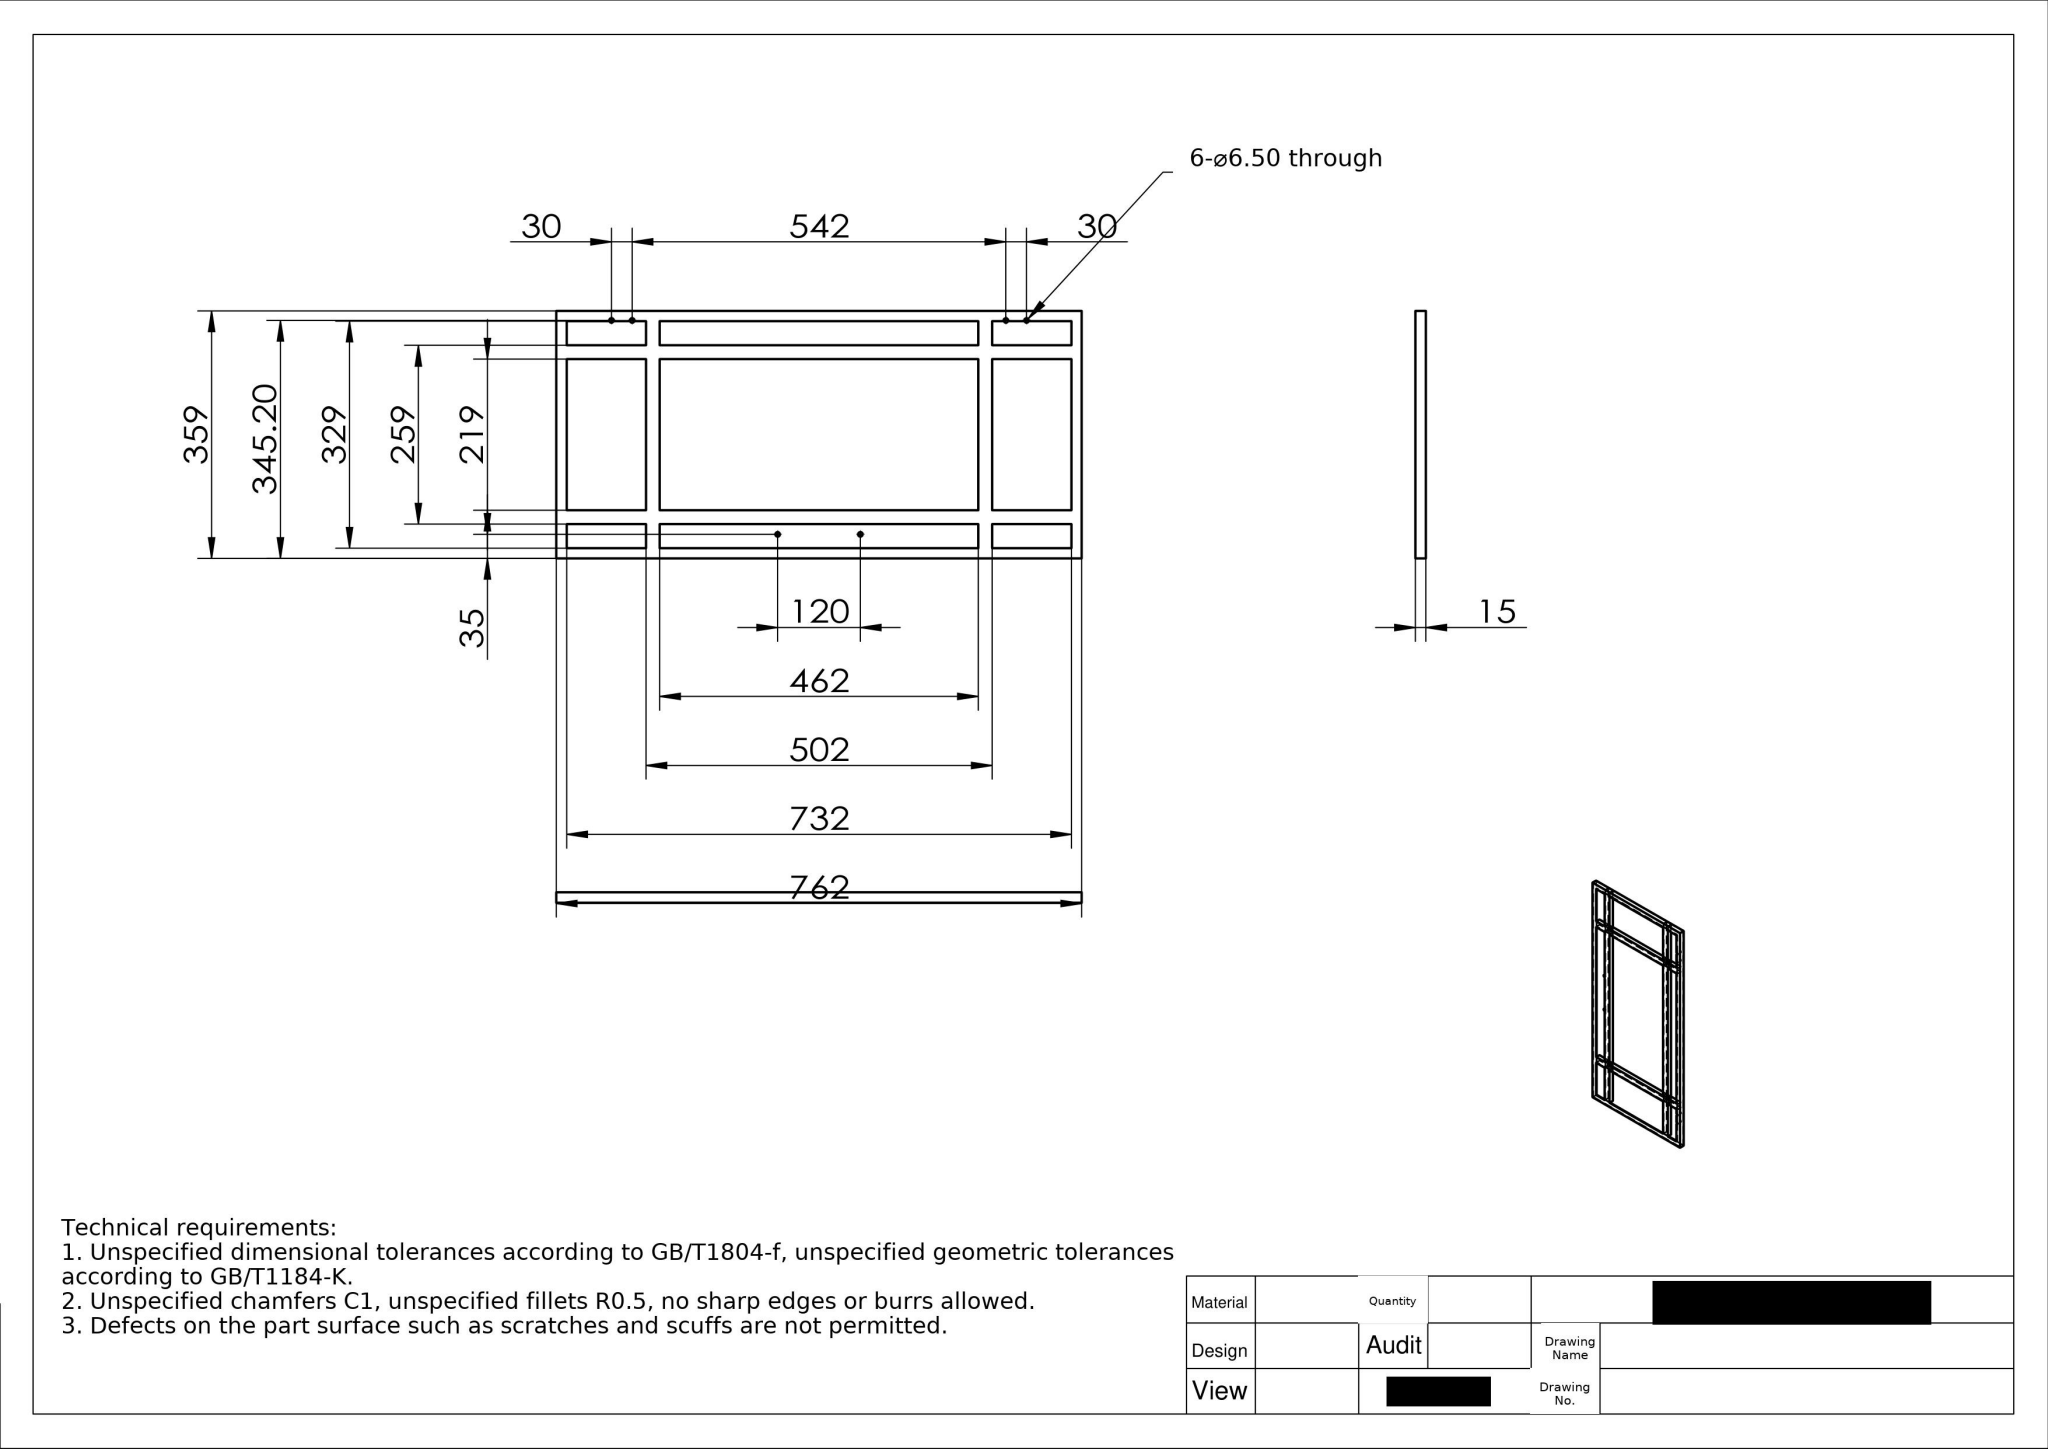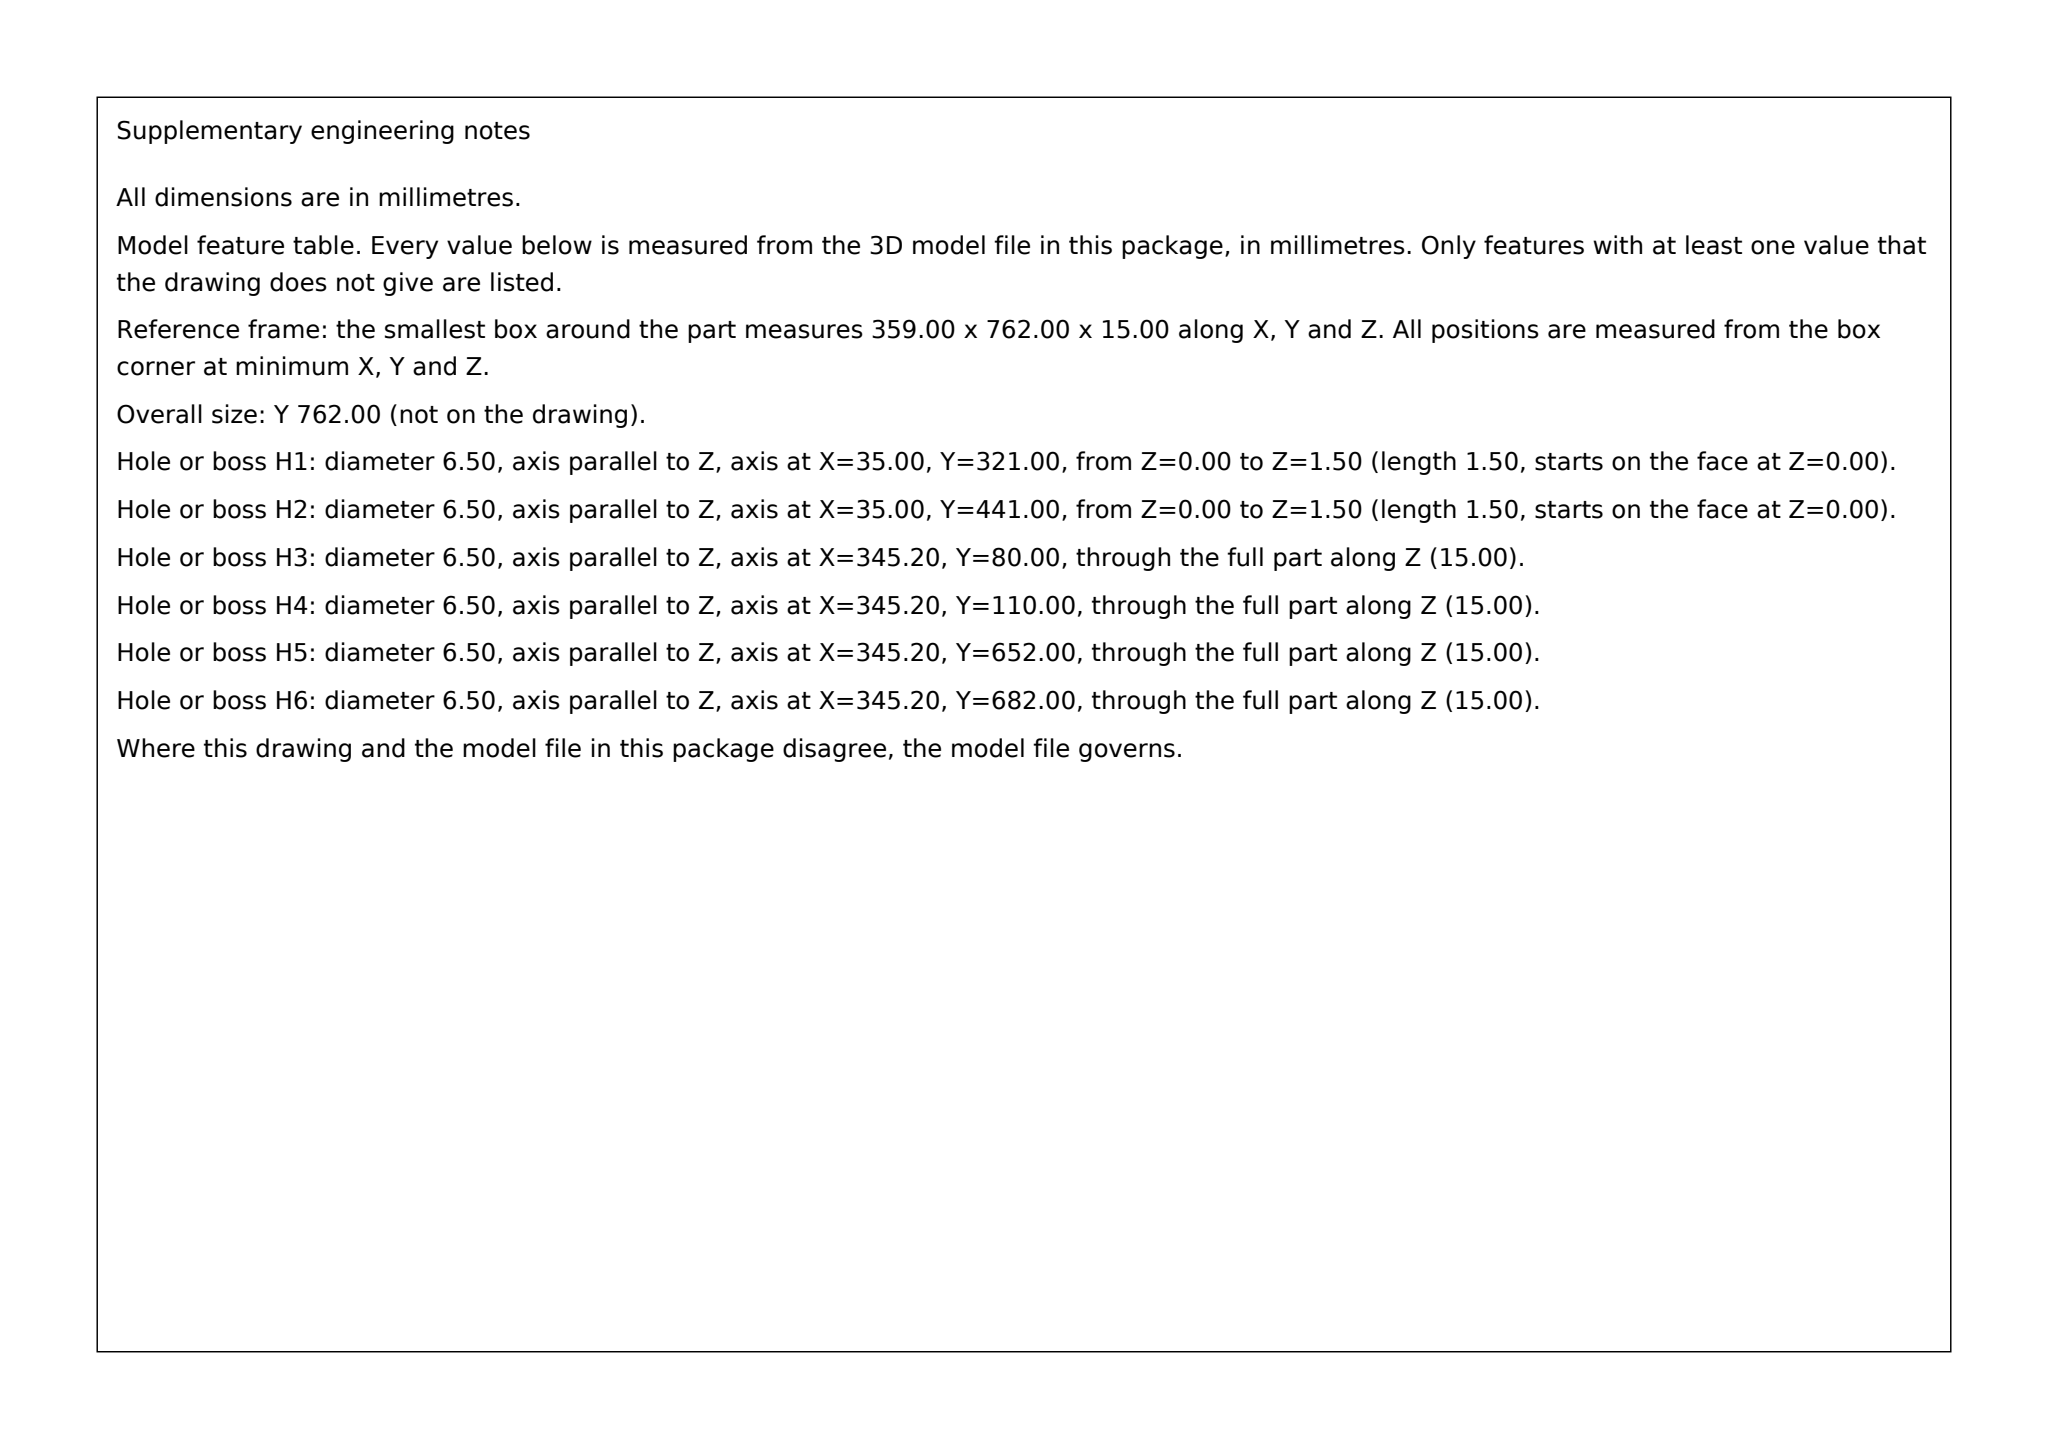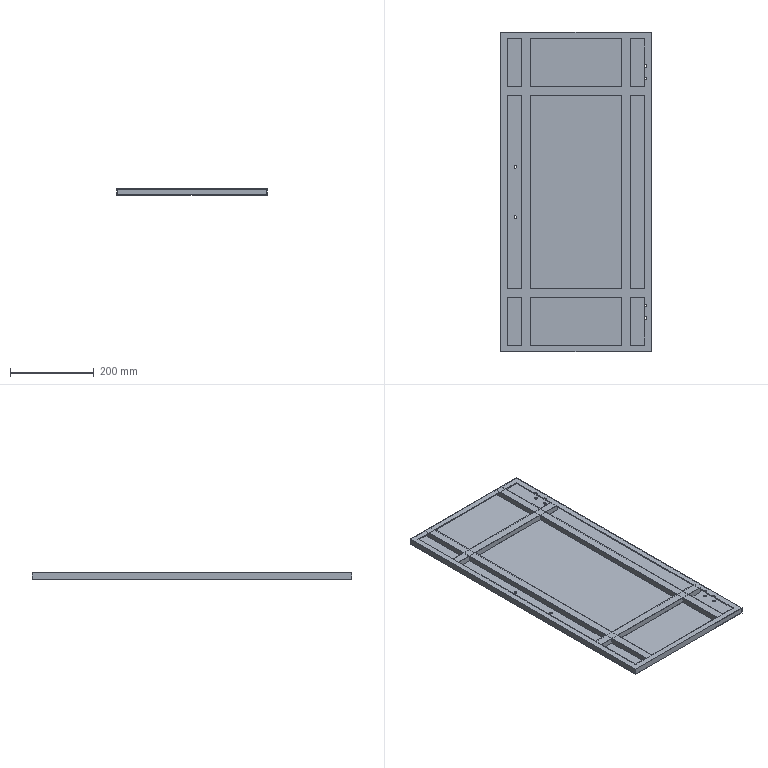Part | SolidWorks | mm | 1 solid | 207 faces | box 359 x 762 x 15 mm | volume 639356 mm3 | plane 191 | cylinder 16 | commonest cylinder face diameters 6.5 x16